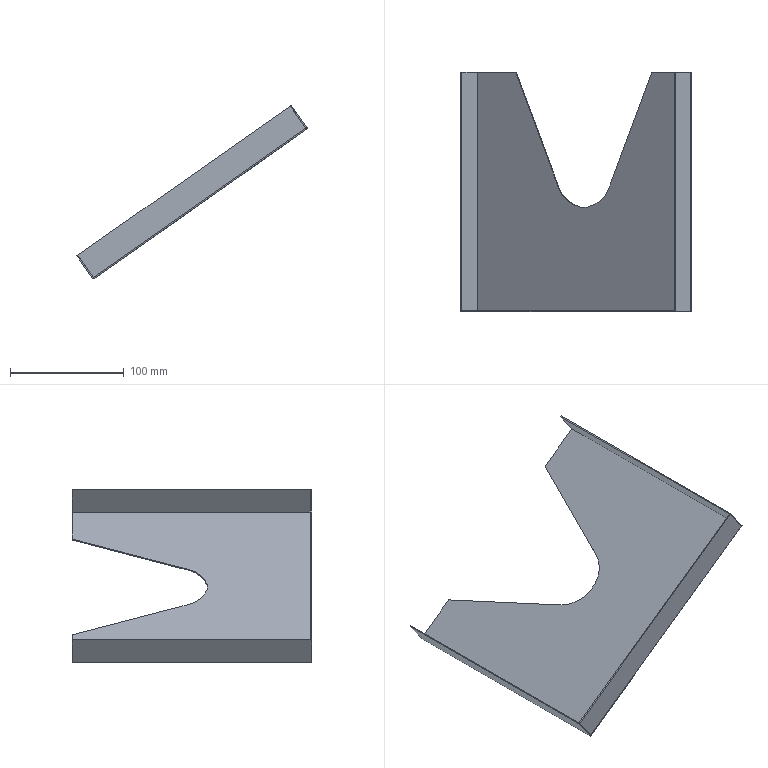Component | SolidWorks | FrontDoorLockHoleWeld-2_DocumentBox-1 | 1 solid | 36 faces | volume 52878 mm3 | plane 29 | cylinder 7 | commonest cylinder face diameters 2.2 x3 0.2 x3 60 x1